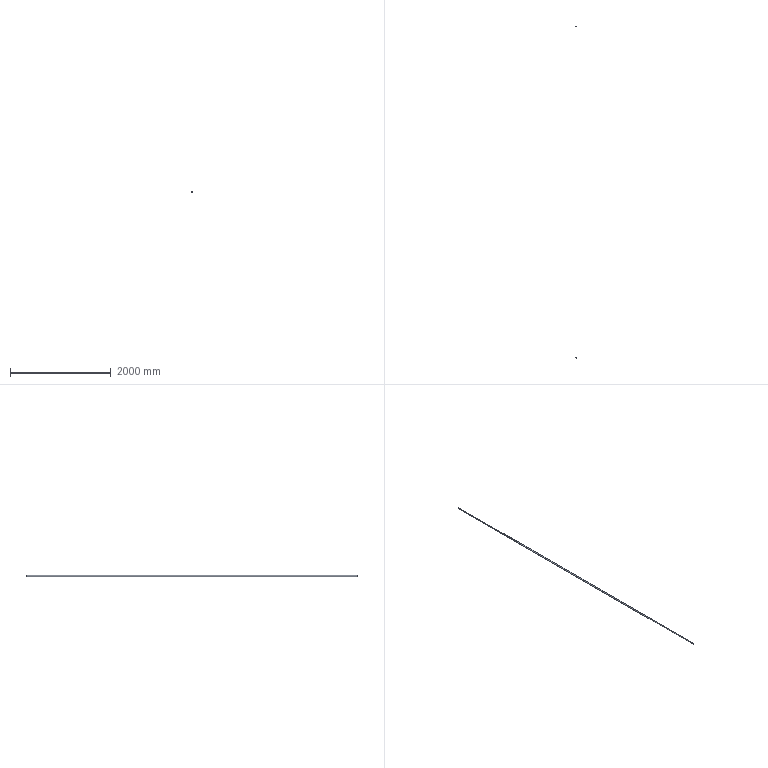Component | NX | 44_4_3 | 1 solid | 4 faces | volume 746329 mm3 | cylinder 2 | plane 2 | commonest cylinder face diameters 20 x1 16 x1